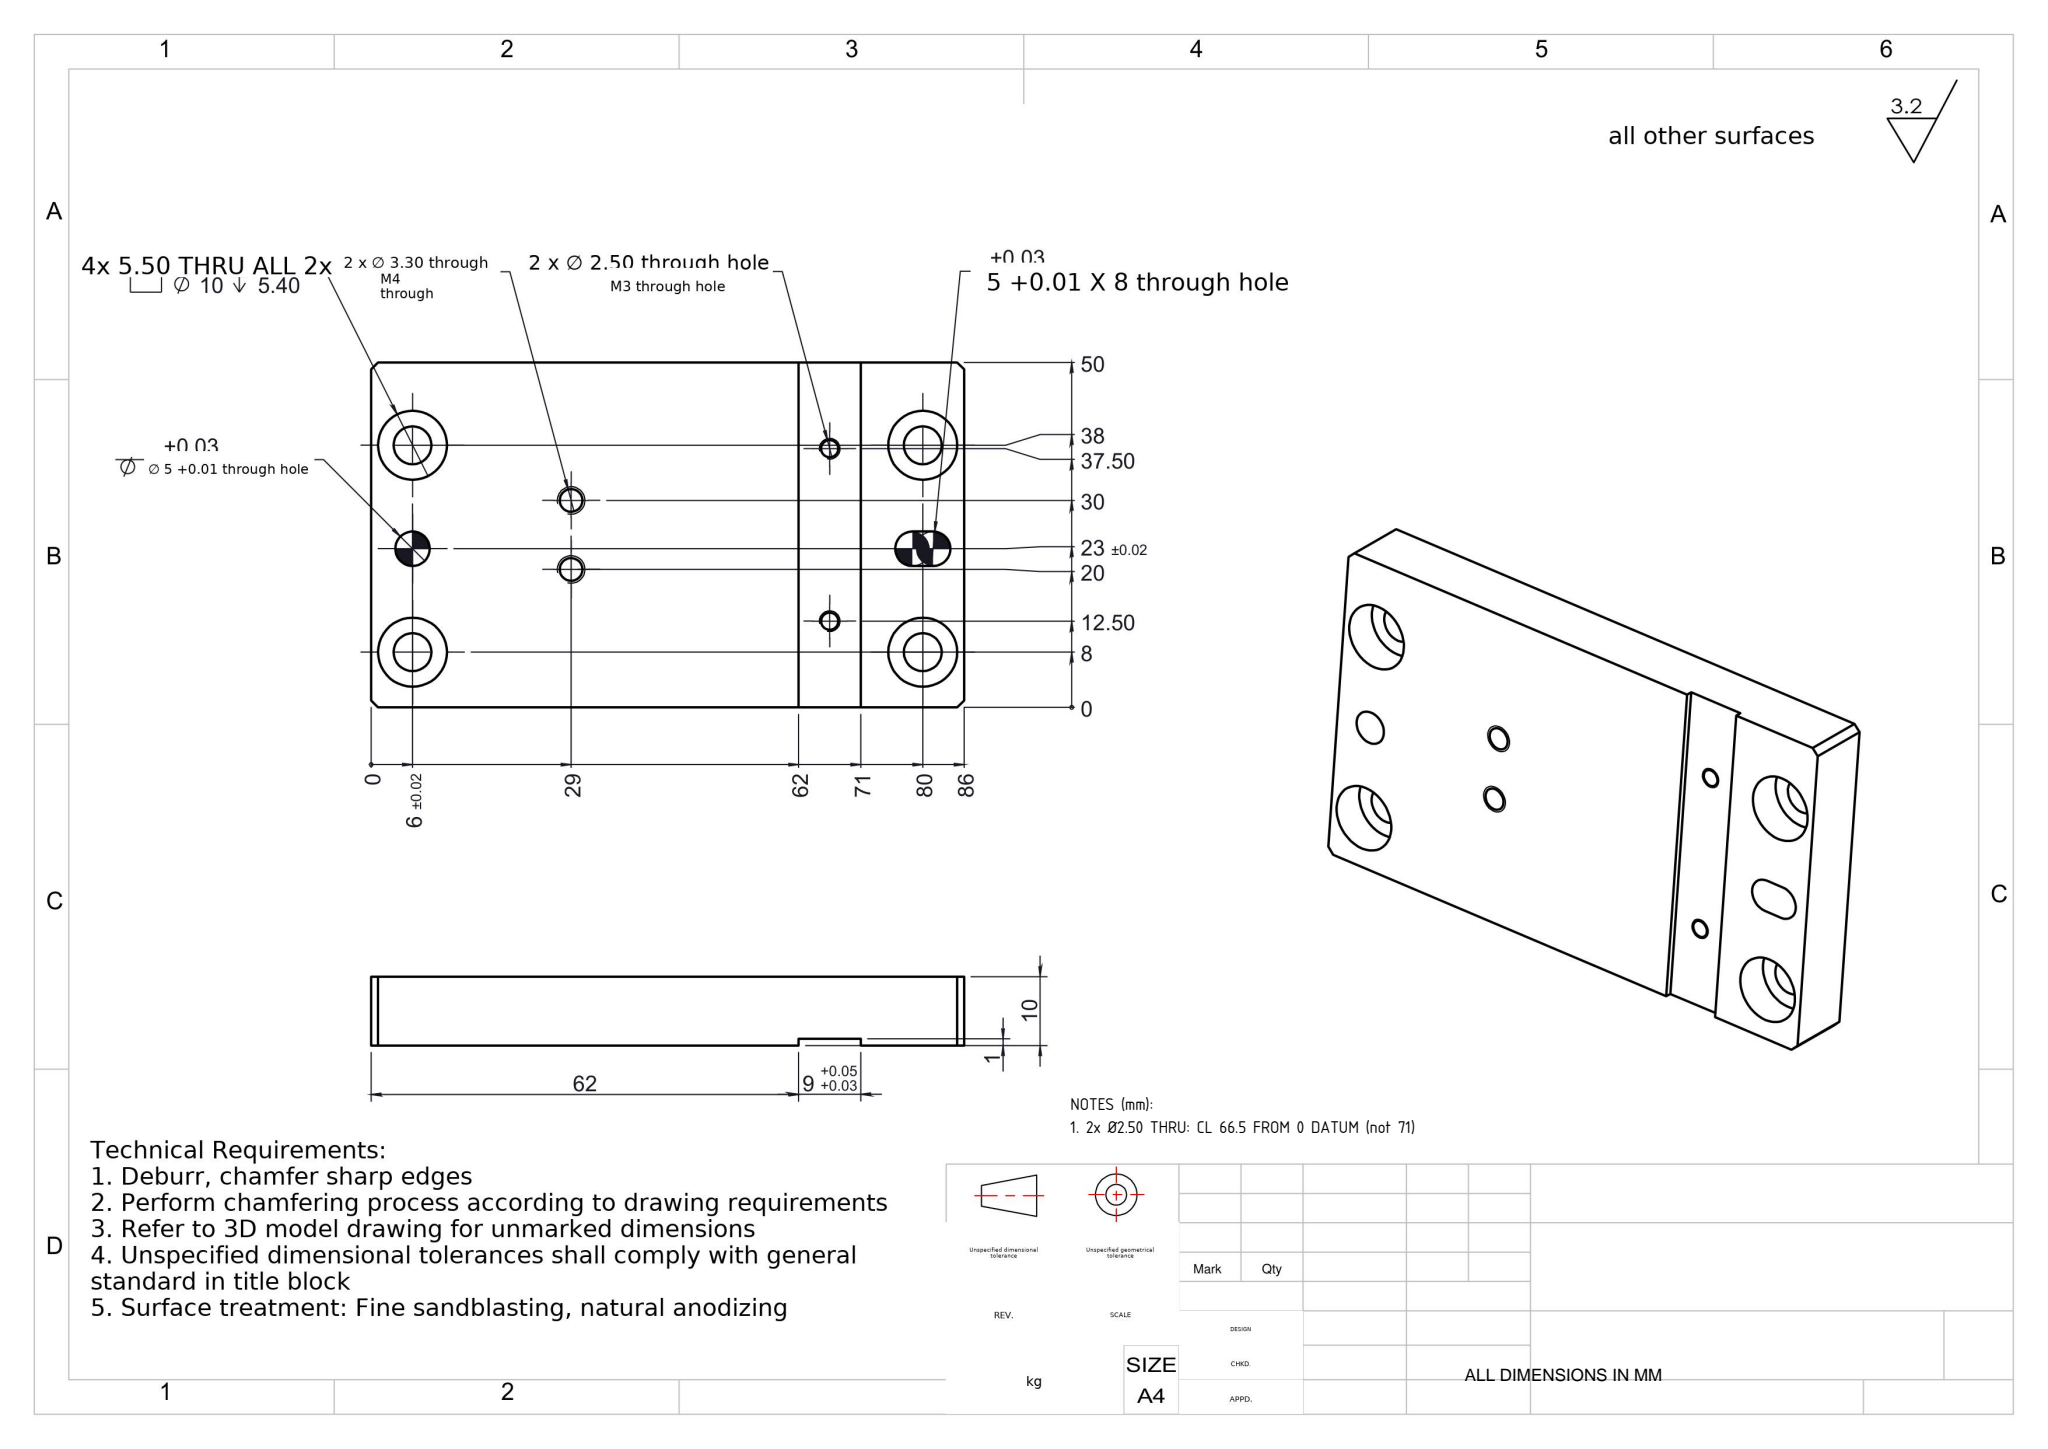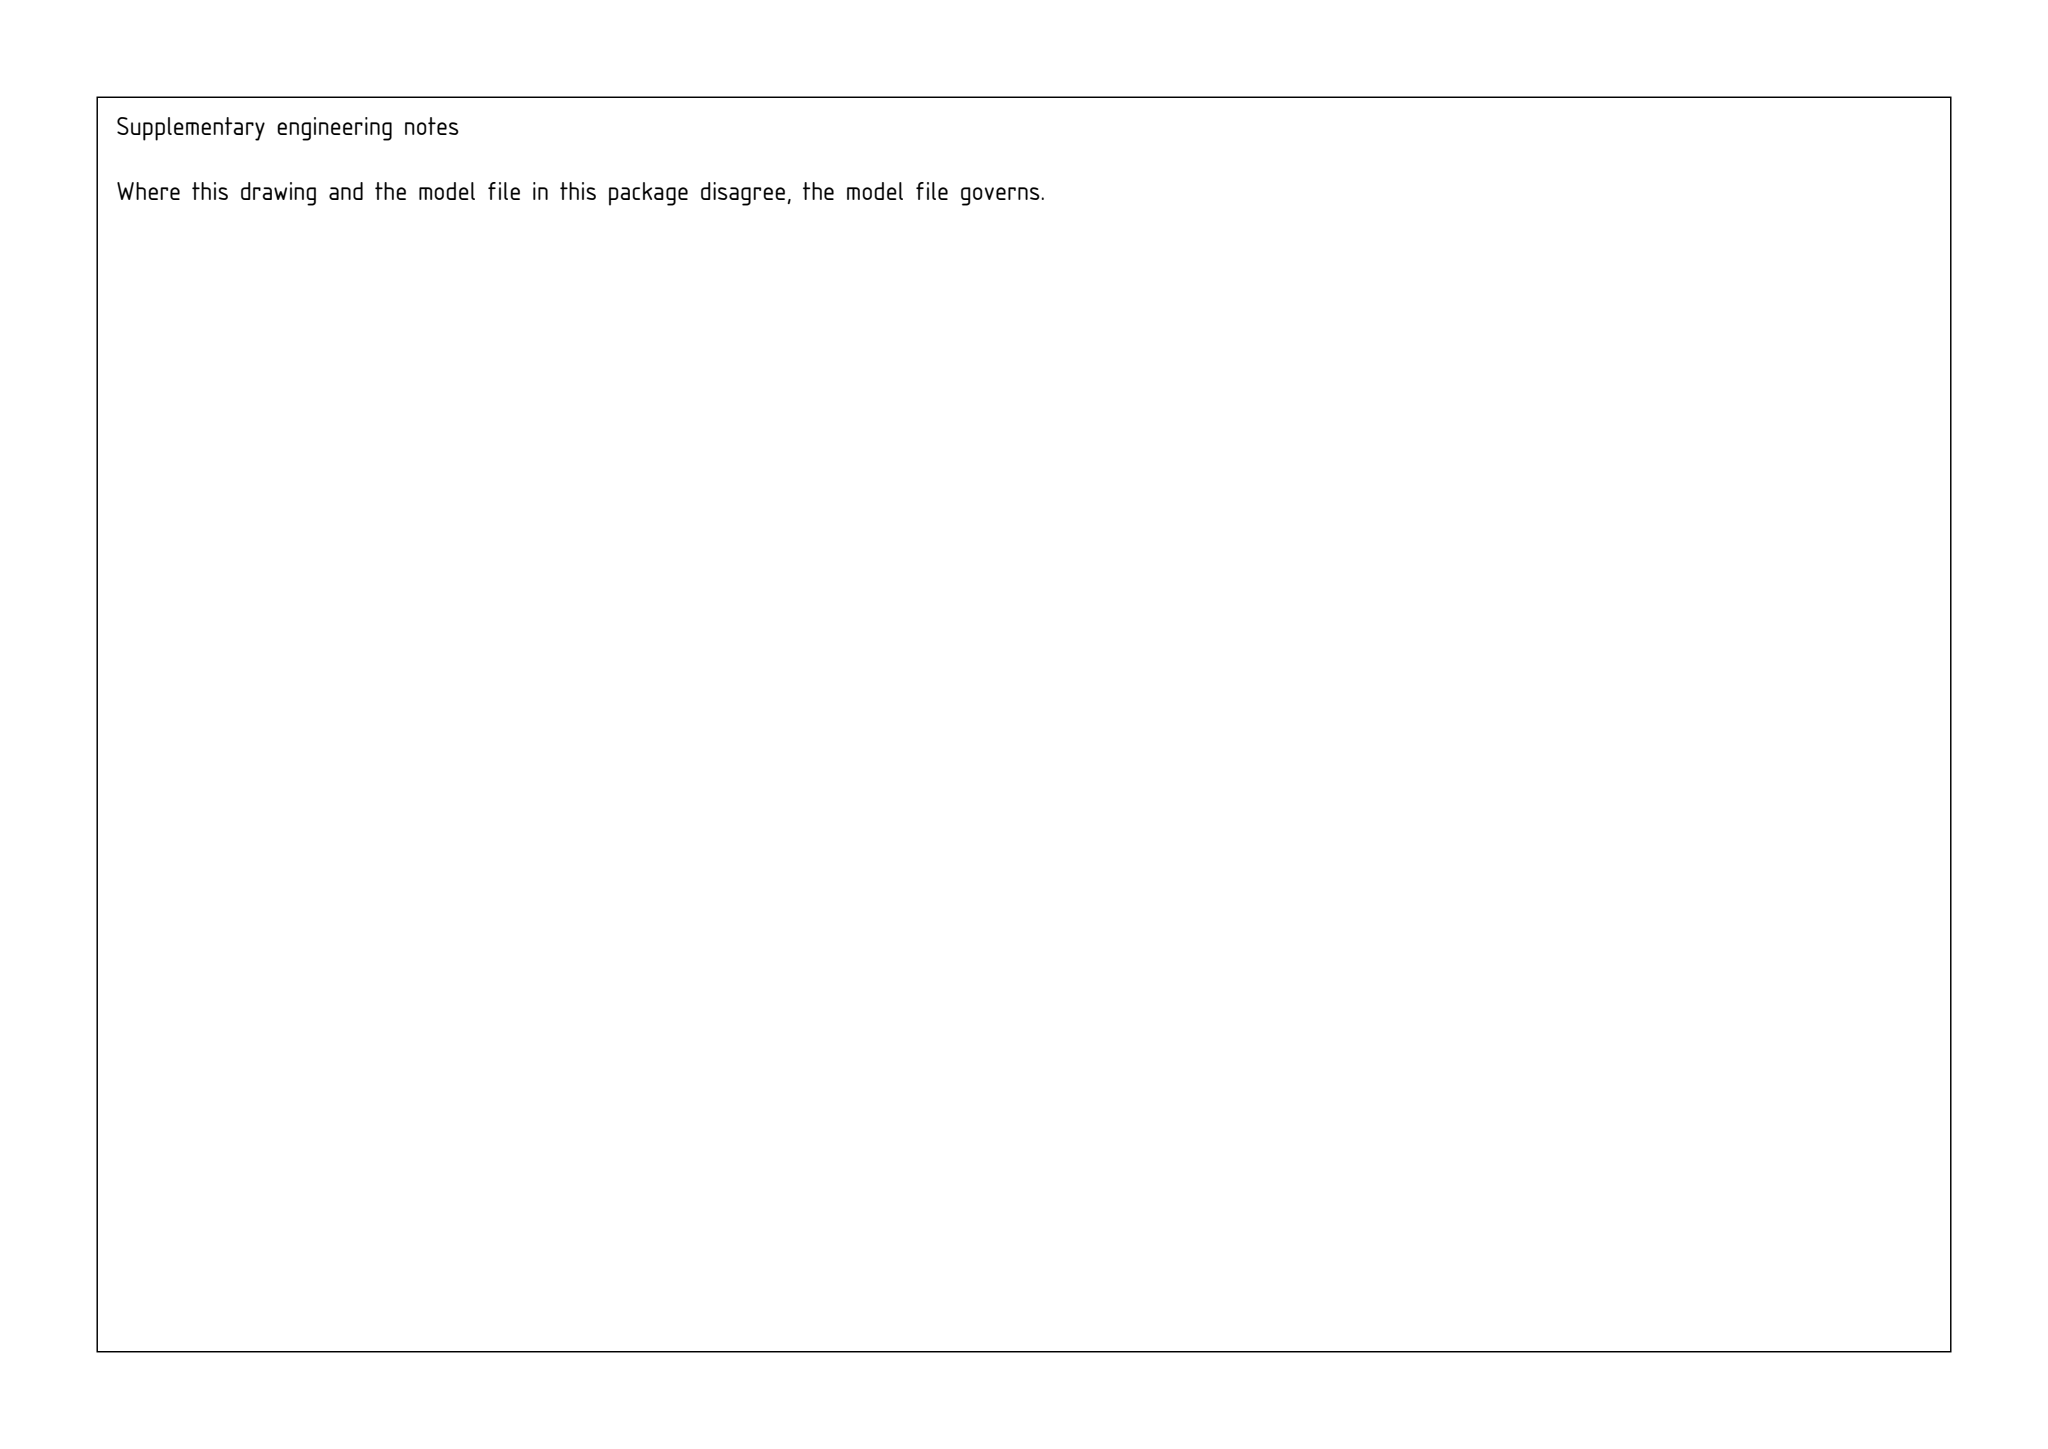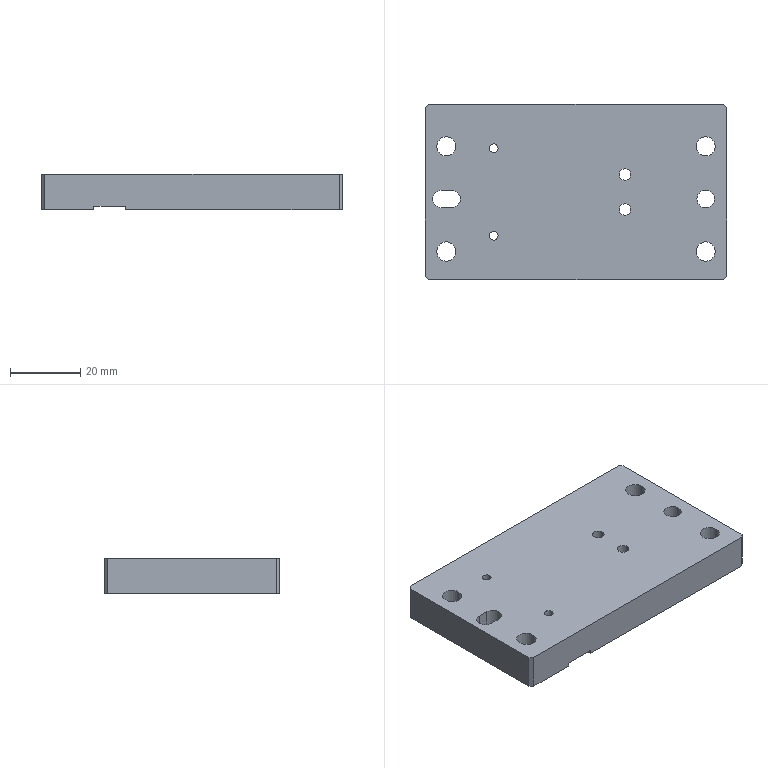Part | SolidWorks | mm | 1 solid | 49 faces | box 86 x 50 x 10 mm | volume 39594 mm3 | cylinder 29 | plane 20 | commonest cylinder face diameters 10 x8 5.5 x8 5 x5 2.5 x4 3.3 x4
Drawing notes:
2x Ø2.50 THRU: CL 66.5 FROM 0 DATUM (not 71) | from the solid: Ø2.5 cyls at x=19.5 from bbox min = 86-19.5 = 66.5 from drawing 0 datum; y=12.5 & 37.5